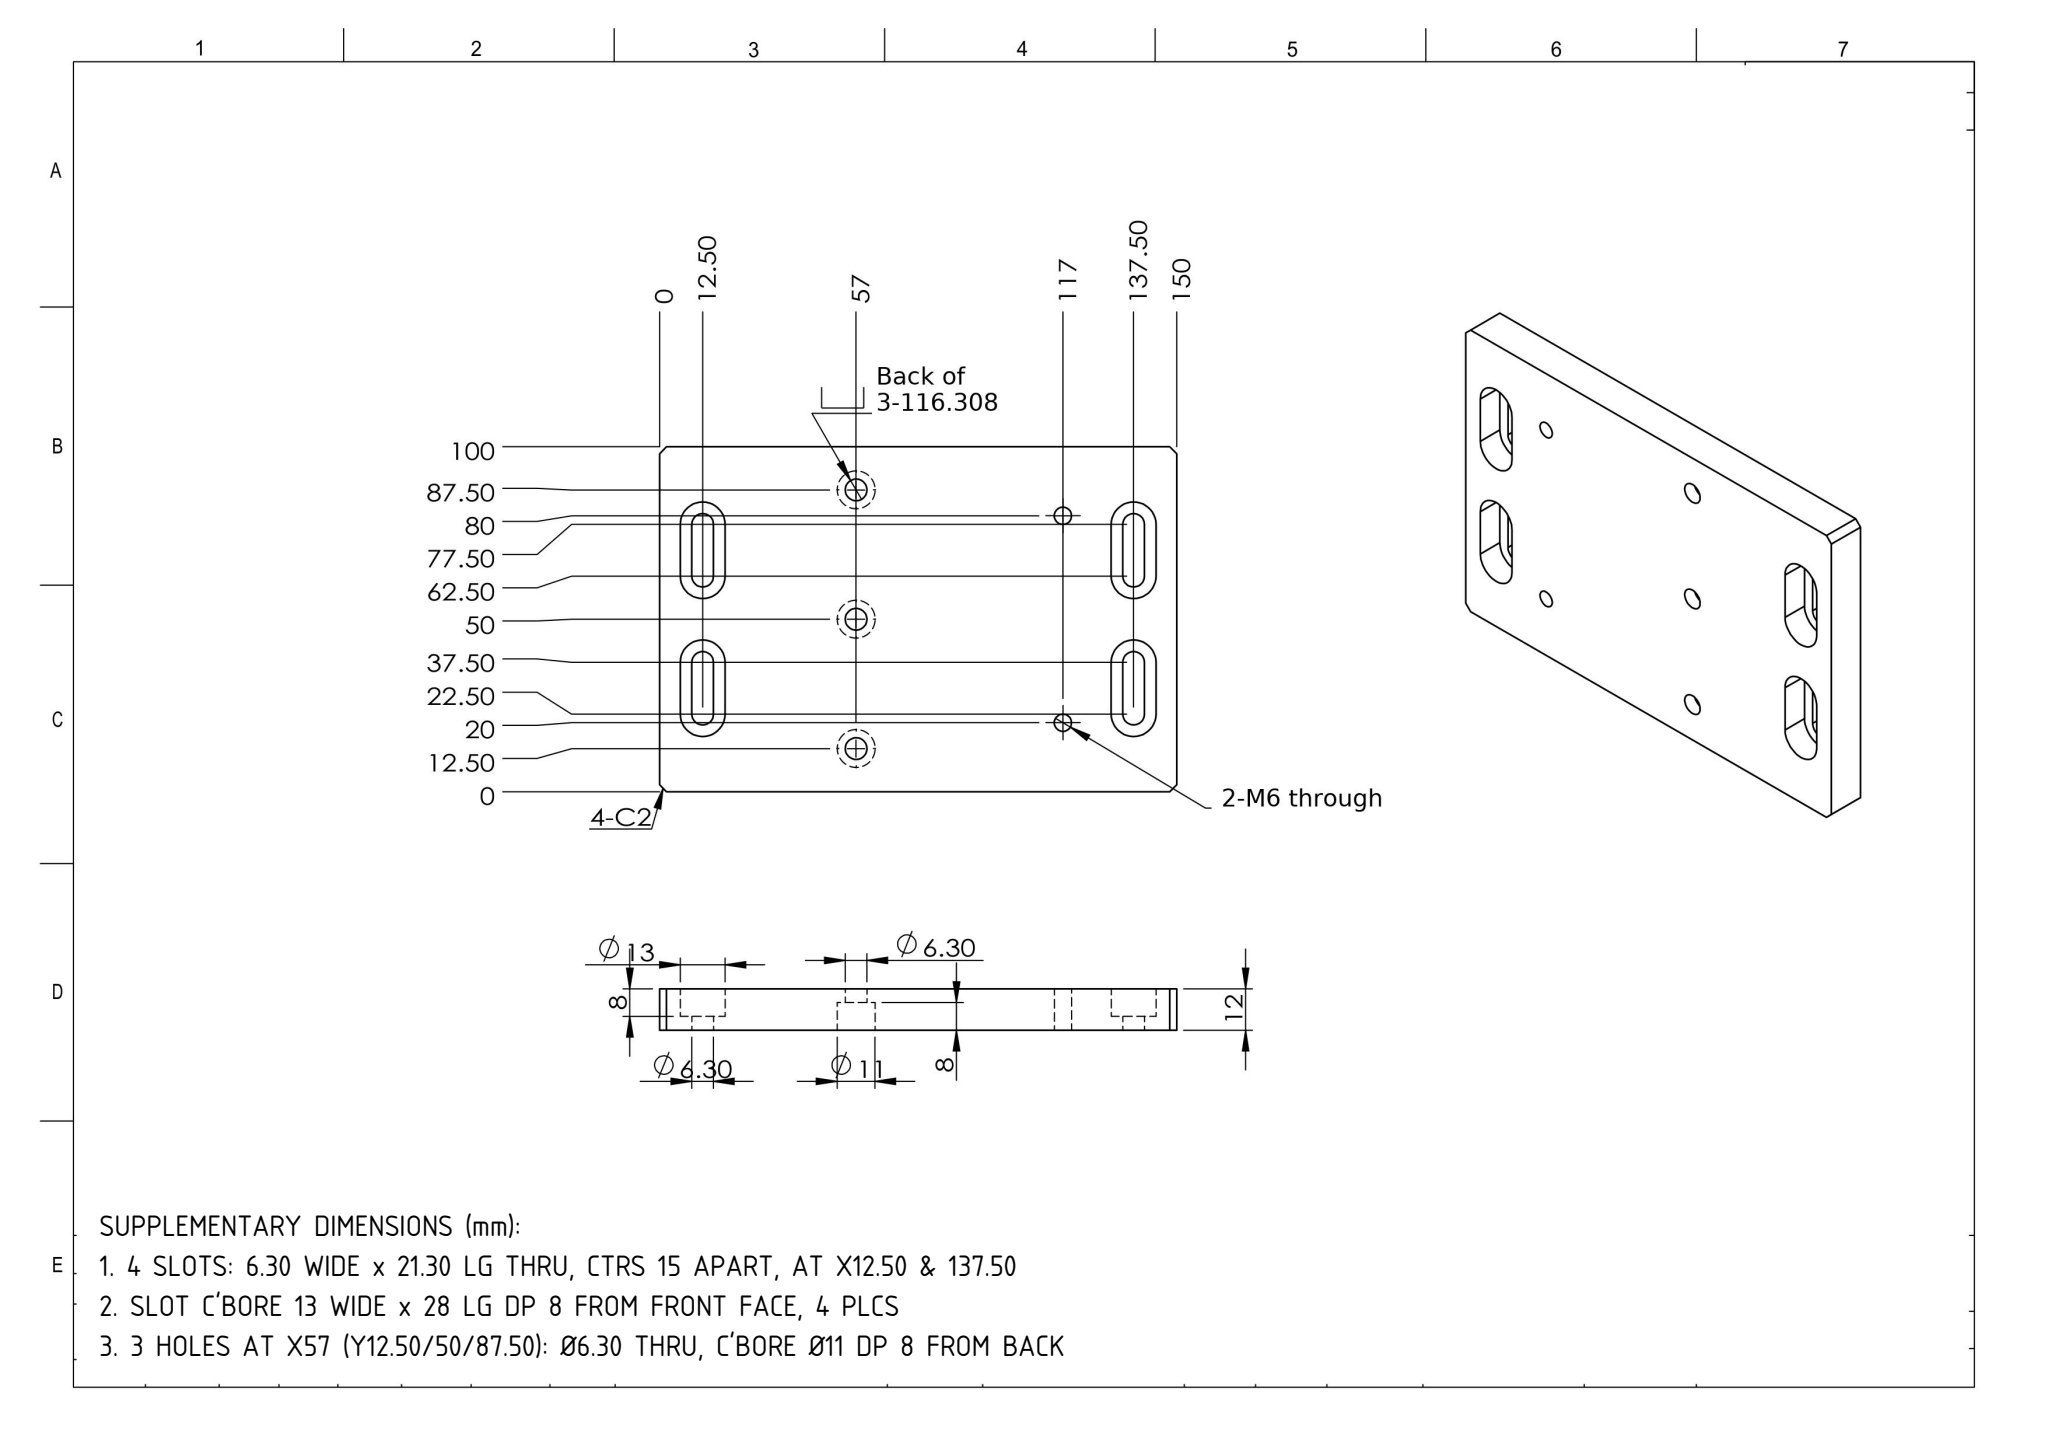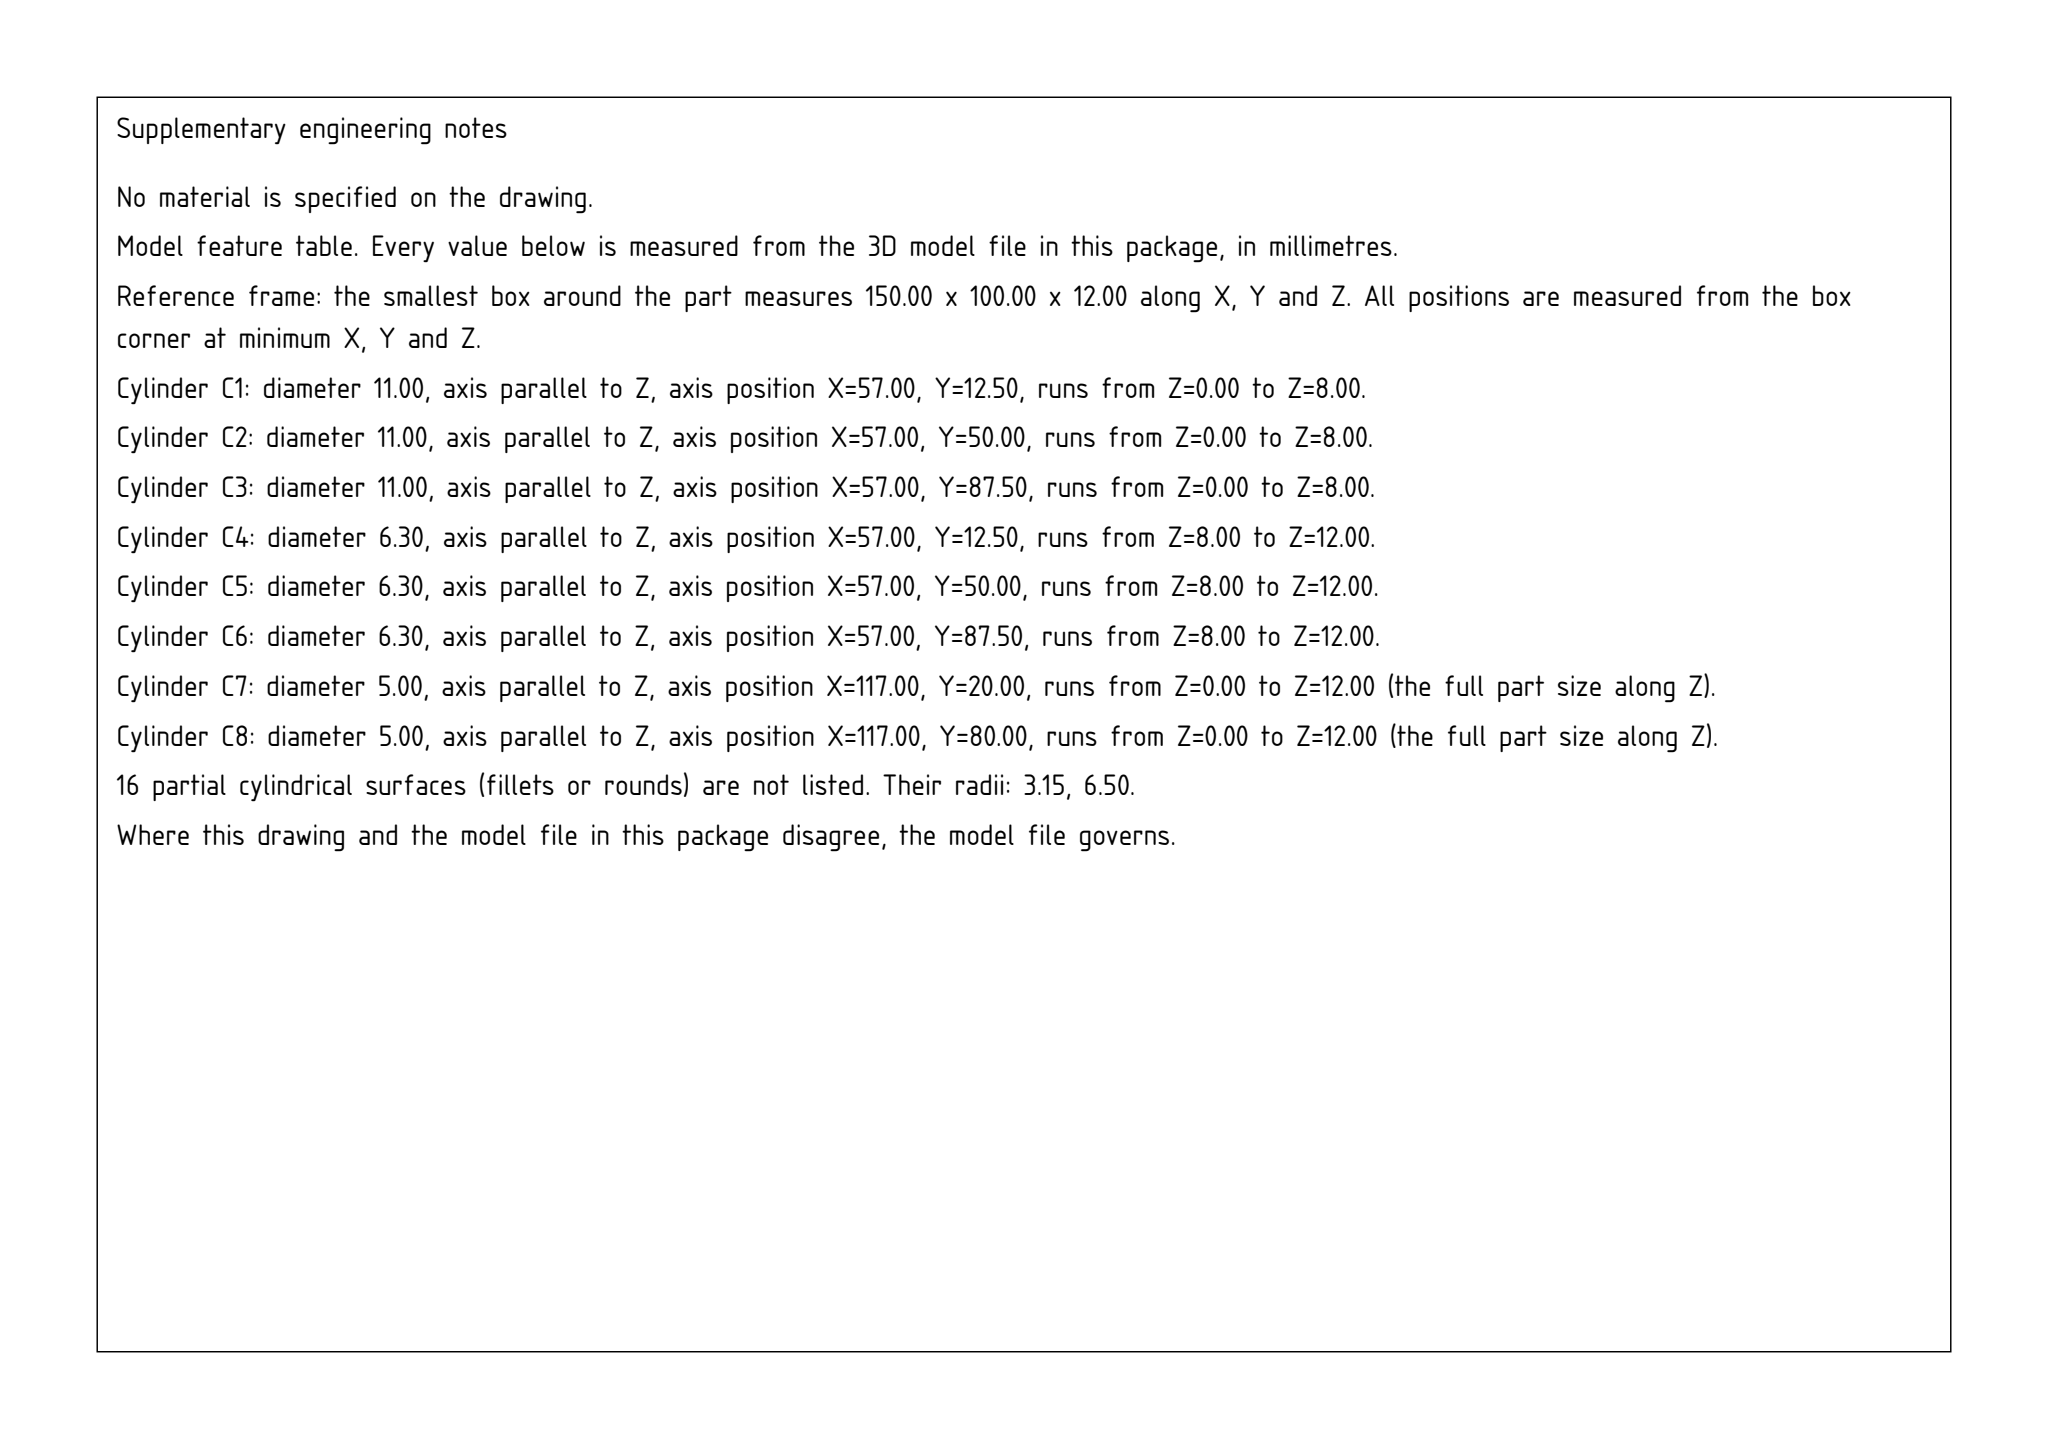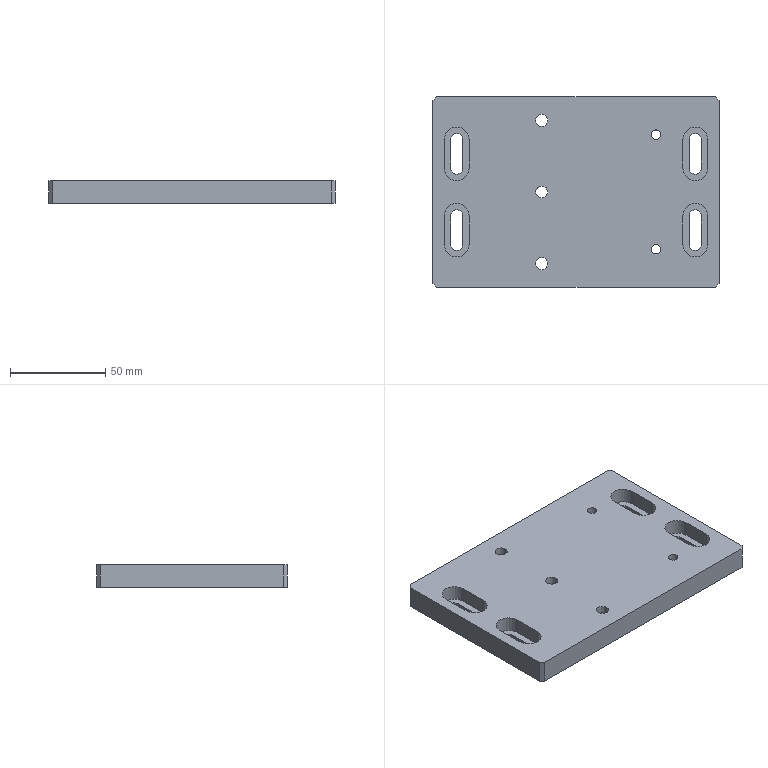Part | SolidWorks | mm | 1 solid | 65 faces | box 150 x 100 x 12 mm | volume 164280 mm3 | plane 33 | cylinder 32 | commonest cylinder face diameters 6.3 x14 13 x8 11 x6 5 x4